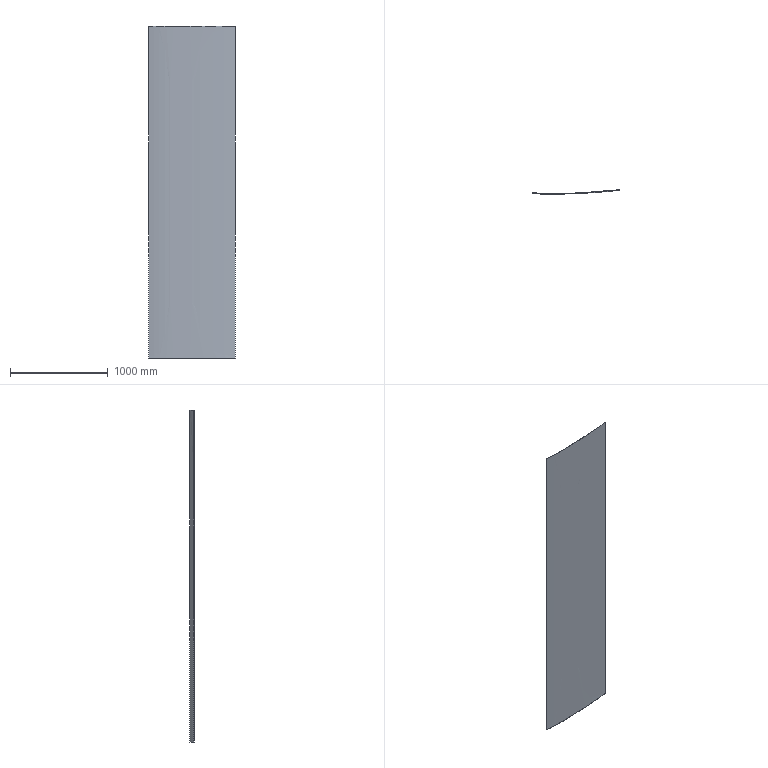Component | NX | SKIN_0_5_LOWER | 1 solid | 6 faces | box 887.13 x 42.02 x 3390 mm | volume 1497879 mm3 | plane 4 | other 2
STEP:
#1=CARTESIAN_POINT('',(0.,0.,0.));
#2=DIRECTION('',(0.,0.,1.));
#3=DIRECTION('',(1.,0.,0.));
#4=AXIS2_PLACEMENT_3D('',#1,#2,#3);
#5=CARTESIAN_POINT('',(5772.888,4104.218,-3390.));
#6=VERTEX_POINT('',#5);
#7=CARTESIAN_POINT('',(5772.824,4103.722,-3390.));
#8=VERTEX_POINT('',#7);
#9=CARTESIAN_POINT('',(5772.888,4104.218,-3390.));
#10=DIRECTION('',(-0.1274,-0.9919,0.));
#11=VECTOR('',#10,1.);
#12=LINE('',#9,#11);
#13=CARTESIAN_POINT('',(5772.888,4104.218,-0.));
#14=DIRECTION('',(0.9919,-0.1274,0.));
#15=DIRECTION('',(0.1274,0.9919,0.));
#16=AXIS2_PLACEMENT_3D('',#13,#14,#15);
#17=PLANE('',#16);
#18=CARTESIAN_POINT('',(0.,-3390.));
#19=DIRECTION('',(-1.,0.));
#20=VECTOR('',#19,1.);
#21=LINE('',#18,#20);
#22=(GEOMETRIC_REPRESENTATION_CONTEXT(2)PARAMETRIC_REPRESENTATION_CONTEXT()REPRESENTATION_CONTEXT('',''));
#23=DEFINITIONAL_REPRESENTATION('',(#21),#22);
#24=PCURVE('',#17,#23);
#25=CARTESIAN_POINT('',(6216.882,4101.421,-3390.));
#26=DIRECTION('',(0.,0.,-1.));
#27=DIRECTION('',(-1.,0.001745,0.));
#28=AXIS2_PLACEMENT_3D('',#25,#26,#27);
#29=PLANE('',#28);
#30=CARTESIAN_POINT('',(443.998,2.021));
#31=DIRECTION('',(0.1256,-0.9921));
#32=VECTOR('',#31,1.);
#33=LINE('',#30,#32);
#34=(GEOMETRIC_REPRESENTATION_CONTEXT(2)PARAMETRIC_REPRESENTATION_CONTEXT()REPRESENTATION_CONTEXT('',''));
#35=DEFINITIONAL_REPRESENTATION('',(#33),#34);
#36=PCURVE('',#29,#35);
#37=SURFACE_CURVE('',#12,(#24,#36),.PCURVE_S1.);
#38=EDGE_CURVE('',#6,#8,#37,.T.);
#39=ORIENTED_EDGE('',*,*,#38,.T.);
#40=CARTESIAN_POINT('',(5772.824,4103.722,-0.));
#41=VERTEX_POINT('',#40);
#42=CARTESIAN_POINT('',(5772.824,4103.722,-0.));
#43=DIRECTION('',(0.,0.,-1.));
#44=VECTOR('',#43,1.);
#45=LINE('',#42,#44);
#46=CARTESIAN_POINT('',(-0.5,0.));
#47=DIRECTION('',(0.,-1.));
#48=VECTOR('',#47,1.);
#49=LINE('',#46,#48);
#50=(GEOMETRIC_REPRESENTATION_CONTEXT(2)PARAMETRIC_REPRESENTATION_CONTEXT()REPRESENTATION_CONTEXT('',''));
#51=DEFINITIONAL_REPRESENTATION('',(#49),#50);
#52=PCURVE('',#17,#51);
#53=CARTESIAN_POINT('',(5772.824,4103.722,0.));
#54=CARTESIAN_POINT('',(5846.499,4094.26,0.));
#55=CARTESIAN_POINT('',(5920.588,4093.032,0.));
#56=CARTESIAN_POINT('',(6013.234,4094.576,0.));
#57=CARTESIAN_POINT('',(6031.765,4095.038,0.));
#58=CARTESIAN_POINT('',(6059.554,4095.829,0.));
#59=CARTESIAN_POINT('',(6068.816,4096.107,0.));
#60=CARTESIAN_POINT('',(6087.337,4096.677,0.));
#61=CARTESIAN_POINT('',(6133.632,4098.144,0.));
#62=CARTESIAN_POINT('',(6179.893,4099.843,0.));
#63=CARTESIAN_POINT('',(6364.839,4107.736,0.));
#64=CARTESIAN_POINT('',(6512.48,4117.559,0.));
#65=CARTESIAN_POINT('',(6659.952,4135.396,0.));
#66=B_SPLINE_CURVE_WITH_KNOTS('',3,(#53,#54,#55,#56,#57,#58,#59,#60,#61,#62,#63,#64,#65),.UNSPECIFIED.,.F.,.F.,(4,2,2,2,1,2,4),(0.,0.25,0.3125,0.3438,0.375,0.5,1.),.UNSPECIFIED.);
#67=DIRECTION('',(0.,0.,-1.));
#68=VECTOR('',#67,1.);
#69=SURFACE_OF_LINEAR_EXTRUSION('',#66,#68);
#70=CARTESIAN_POINT('',(-0.,0.));
#71=DIRECTION('',(0.,1.));
#72=VECTOR('',#71,1.);
#73=LINE('',#70,#72);
#74=(GEOMETRIC_REPRESENTATION_CONTEXT(2)PARAMETRIC_REPRESENTATION_CONTEXT()REPRESENTATION_CONTEXT('',''));
#75=DEFINITIONAL_REPRESENTATION('',(#73),#74);
#76=PCURVE('',#69,#75);
#77=SURFACE_CURVE('',#45,(#52,#76),.PCURVE_S1.);
#78=EDGE_CURVE('',#41,#8,#77,.T.);
#79=ORIENTED_EDGE('',*,*,#78,.F.);
#80=CARTESIAN_POINT('',(5772.888,4104.218,-0.));
#81=VERTEX_POINT('',#80);
#82=CARTESIAN_POINT('',(5772.888,4104.218,-0.));
#83=DIRECTION('',(-0.1274,-0.9919,0.));
#84=VECTOR('',#83,1.);
#85=LINE('',#82,#84);
#86=CARTESIAN_POINT('',(0.,0.));
#87=DIRECTION('',(-1.,0.));
#88=VECTOR('',#87,1.);
#89=LINE('',#86,#88);
#90=(GEOMETRIC_REPRESENTATION_CONTEXT(2)PARAMETRIC_REPRESENTATION_CONTEXT()REPRESENTATION_CONTEXT('',''));
#91=DEFINITIONAL_REPRESENTATION('',(#89),#90);
#92=PCURVE('',#17,#91);
#93=CARTESIAN_POINT('',(6216.882,4101.421,0.));
#94=DIRECTION('',(0.,0.,-1.));
#95=DIRECTION('',(-1.,0.001745,0.));
#96=AXIS2_PLACEMENT_3D('',#93,#94,#95);
#97=PLANE('',#96);
#98=CARTESIAN_POINT('',(443.998,2.021));
#99=DIRECTION('',(0.1256,-0.9921));
#100=VECTOR('',#99,1.);
#101=LINE('',#98,#100);
#102=(GEOMETRIC_REPRESENTATION_CONTEXT(2)PARAMETRIC_REPRESENTATION_CONTEXT()REPRESENTATION_CONTEXT('',''));
#103=DEFINITIONAL_REPRESENTATION('',(#101),#102);
#104=PCURVE('',#97,#103);
#105=SURFACE_CURVE('',#85,(#92,#104),.PCURVE_S1.);
#106=EDGE_CURVE('',#81,#41,#105,.T.);
#107=ORIENTED_EDGE('',*,*,#106,.F.);
#108=CARTESIAN_POINT('',(5772.888,4104.218,-0.));
#109=DIRECTION('',(0.,0.,-1.));
#110=VECTOR('',#109,1.);
#111=LINE('',#108,#110);
#112=CARTESIAN_POINT('',(0.,0.));
#113=DIRECTION('',(0.,-1.));
#114=VECTOR('',#113,1.);
#115=LINE('',#112,#114);
#116=(GEOMETRIC_REPRESENTATION_CONTEXT(2)PARAMETRIC_REPRESENTATION_CONTEXT()REPRESENTATION_CONTEXT('',''));
#117=DEFINITIONAL_REPRESENTATION('',(#115),#116);
#118=PCURVE('',#17,#117);
#119=CARTESIAN_POINT('',(6659.892,4135.892,-0.));
#120=CARTESIAN_POINT('',(6463.767,4112.17,-0.));
#121=CARTESIAN_POINT('',(6168.395,4097.815,-0.));
#122=CARTESIAN_POINT('',(5871.551,4091.547,-0.));
#123=CARTESIAN_POINT('',(5772.888,4104.218,-0.));
#124=B_SPLINE_CURVE_WITH_KNOTS('',3,(#119,#120,#121,#122,#123),.UNSPECIFIED.,.F.,.F.,(4,1,4),(0.,0.665,1.),.UNSPECIFIED.);
#125=DIRECTION('',(0.,0.,-1.));
#126=VECTOR('',#125,1.);
#127=SURFACE_OF_LINEAR_EXTRUSION('',#124,#126);
#128=CARTESIAN_POINT('',(1.,0.));
#129=DIRECTION('',(-0.,1.));
#130=VECTOR('',#129,1.);
#131=LINE('',#128,#130);
#132=(GEOMETRIC_REPRESENTATION_CONTEXT(2)PARAMETRIC_REPRESENTATION_CONTEXT()REPRESENTATION_CONTEXT('',''));
#133=DEFINITIONAL_REPRESENTATION('',(#131),#132);
#134=PCURVE('',#127,#133);
#135=SURFACE_CURVE('',#111,(#118,#134),.PCURVE_S1.);
#136=EDGE_CURVE('',#81,#6,#135,.T.);
#137=ORIENTED_EDGE('',*,*,#136,.T.);
#138=EDGE_LOOP('',(#39,#79,#107,#137));
#139=FACE_BOUND('',#138,.T.);
#140=ADVANCED_FACE('',(#139),#17,.F.);
#141=ORIENTED_EDGE('',*,*,#78,.F.);
#142=CARTESIAN_POINT('',(6659.952,4135.396,0.));
#143=VERTEX_POINT('',#142);
#144=CARTESIAN_POINT('',(5772.824,4103.722,0.));
#145=CARTESIAN_POINT('',(5846.499,4094.26,0.));
#146=CARTESIAN_POINT('',(5920.588,4093.032,0.));
#147=CARTESIAN_POINT('',(6013.234,4094.576,0.));
#148=CARTESIAN_POINT('',(6031.765,4095.038,0.));
#149=CARTESIAN_POINT('',(6059.554,4095.829,0.));
#150=CARTESIAN_POINT('',(6068.816,4096.107,0.));
#151=CARTESIAN_POINT('',(6087.337,4096.677,0.));
#152=CARTESIAN_POINT('',(6133.632,4098.144,0.));
#153=CARTESIAN_POINT('',(6179.893,4099.843,0.));
#154=CARTESIAN_POINT('',(6364.839,4107.736,0.));
#155=CARTESIAN_POINT('',(6512.48,4117.559,0.));
#156=CARTESIAN_POINT('',(6659.952,4135.396,0.));
#157=B_SPLINE_CURVE_WITH_KNOTS('',3,(#144,#145,#146,#147,#148,#149,#150,#151,#152,#153,#154,#155,#156),.UNSPECIFIED.,.F.,.F.,(4,2,2,2,1,2,4),(0.,0.25,0.3125,0.3438,0.375,0.5,1.),.UNSPECIFIED.);
#158=CARTESIAN_POINT('',(-0.,0.));
#159=DIRECTION('',(1.,0.));
#160=VECTOR('',#159,1.);
#161=LINE('',#158,#160);
#162=(GEOMETRIC_REPRESENTATION_CONTEXT(2)PARAMETRIC_REPRESENTATION_CONTEXT()REPRESENTATION_CONTEXT('',''));
#163=DEFINITIONAL_REPRESENTATION('',(#161),#162);
#164=PCURVE('',#69,#163);
#165=CARTESIAN_POINT('',(444.061,1.525));
#166=CARTESIAN_POINT('',(370.371,-7.808));
#167=CARTESIAN_POINT('',(296.279,-8.907));
#168=CARTESIAN_POINT('',(203.636,-7.201));
#169=CARTESIAN_POINT('',(185.106,-6.706));
#170=CARTESIAN_POINT('',(157.318,-5.867));
#171=CARTESIAN_POINT('',(148.057,-5.573));
#172=CARTESIAN_POINT('',(129.537,-4.97));
#173=CARTESIAN_POINT('',(83.244,-3.423));
#174=CARTESIAN_POINT('',(36.986,-1.643));
#175=CARTESIAN_POINT('',(-147.945,6.572));
#176=CARTESIAN_POINT('',(-295.569,16.653));
#177=CARTESIAN_POINT('',(-443.01,34.747));
#178=B_SPLINE_CURVE_WITH_KNOTS('',3,(#165,#166,#167,#168,#169,#170,#171,#172,#173,#174,#175,#176,#177),.UNSPECIFIED.,.F.,.F.,(4,2,2,2,1,2,4),(0.,0.25,0.3125,0.3438,0.375,0.5,1.),.UNSPECIFIED.);
#179=(GEOMETRIC_REPRESENTATION_CONTEXT(2)PARAMETRIC_REPRESENTATION_CONTEXT()REPRESENTATION_CONTEXT('',''));
#180=DEFINITIONAL_REPRESENTATION('',(#178),#179);
#181=PCURVE('',#97,#180);
#182=SURFACE_CURVE('',#157,(#164,#181),.PCURVE_S1.);
#183=EDGE_CURVE('',#41,#143,#182,.T.);
#184=ORIENTED_EDGE('',*,*,#183,.T.);
#185=CARTESIAN_POINT('',(6659.952,4135.396,-3390.));
#186=VERTEX_POINT('',#185);
#187=CARTESIAN_POINT('',(6659.952,4135.396,0.));
#188=DIRECTION('',(0.,0.,-1.));
#189=VECTOR('',#188,1.);
#190=LINE('',#187,#189);
#191=CARTESIAN_POINT('',(1.,0.));
#192=DIRECTION('',(0.,1.));
#193=VECTOR('',#192,1.);
#194=LINE('',#191,#193);
#195=(GEOMETRIC_REPRESENTATION_CONTEXT(2)PARAMETRIC_REPRESENTATION_CONTEXT()REPRESENTATION_CONTEXT('',''));
#196=DEFINITIONAL_REPRESENTATION('',(#194),#195);
#197=PCURVE('',#69,#196);
#198=CARTESIAN_POINT('',(6659.952,4135.396,-0.));
#199=DIRECTION('',(-0.9928,-0.1201,0.));
#200=DIRECTION('',(0.1201,-0.9928,0.));
#201=AXIS2_PLACEMENT_3D('',#198,#199,#200);
#202=PLANE('',#201);
#203=CARTESIAN_POINT('',(0.,0.));
#204=DIRECTION('',(0.,-1.));
#205=VECTOR('',#204,1.);
#206=LINE('',#203,#205);
#207=(GEOMETRIC_REPRESENTATION_CONTEXT(2)PARAMETRIC_REPRESENTATION_CONTEXT()REPRESENTATION_CONTEXT('',''));
#208=DEFINITIONAL_REPRESENTATION('',(#206),#207);
#209=PCURVE('',#202,#208);
#210=SURFACE_CURVE('',#190,(#197,#209),.PCURVE_S1.);
#211=EDGE_CURVE('',#143,#186,#210,.T.);
#212=ORIENTED_EDGE('',*,*,#211,.T.);
#213=CARTESIAN_POINT('',(5772.824,4103.722,-3390.));
#214=CARTESIAN_POINT('',(5846.499,4094.26,-3390.));
#215=CARTESIAN_POINT('',(5920.588,4093.032,-3390.));
#216=CARTESIAN_POINT('',(6013.234,4094.576,-3390.));
#217=CARTESIAN_POINT('',(6031.765,4095.038,-3390.));
#218=CARTESIAN_POINT('',(6059.554,4095.829,-3390.));
#219=CARTESIAN_POINT('',(6068.816,4096.107,-3390.));
#220=CARTESIAN_POINT('',(6087.337,4096.677,-3390.));
#221=CARTESIAN_POINT('',(6133.632,4098.144,-3390.));
#222=CARTESIAN_POINT('',(6179.893,4099.843,-3390.));
#223=CARTESIAN_POINT('',(6364.839,4107.736,-3390.));
#224=CARTESIAN_POINT('',(6512.48,4117.559,-3390.));
#225=CARTESIAN_POINT('',(6659.952,4135.396,-3390.));
#226=B_SPLINE_CURVE_WITH_KNOTS('',3,(#213,#214,#215,#216,#217,#218,#219,#220,#221,#222,#223,#224,#225),.UNSPECIFIED.,.F.,.F.,(4,2,2,2,1,2,4),(0.,0.25,0.3125,0.3438,0.375,0.5,1.),.UNSPECIFIED.);
#227=CARTESIAN_POINT('',(0.,3390.));
#228=DIRECTION('',(1.,0.));
#229=VECTOR('',#228,1.);
#230=LINE('',#227,#229);
#231=(GEOMETRIC_REPRESENTATION_CONTEXT(2)PARAMETRIC_REPRESENTATION_CONTEXT()REPRESENTATION_CONTEXT('',''));
#232=DEFINITIONAL_REPRESENTATION('',(#230),#231);
#233=PCURVE('',#69,#232);
#234=CARTESIAN_POINT('',(444.061,1.525));
#235=CARTESIAN_POINT('',(370.371,-7.808));
#236=CARTESIAN_POINT('',(296.279,-8.907));
#237=CARTESIAN_POINT('',(203.636,-7.201));
#238=CARTESIAN_POINT('',(185.106,-6.706));
#239=CARTESIAN_POINT('',(157.318,-5.867));
#240=CARTESIAN_POINT('',(148.057,-5.573));
#241=CARTESIAN_POINT('',(129.537,-4.97));
#242=CARTESIAN_POINT('',(83.244,-3.423));
#243=CARTESIAN_POINT('',(36.986,-1.643));
#244=CARTESIAN_POINT('',(-147.945,6.572));
#245=CARTESIAN_POINT('',(-295.569,16.653));
#246=CARTESIAN_POINT('',(-443.01,34.747));
#247=B_SPLINE_CURVE_WITH_KNOTS('',3,(#234,#235,#236,#237,#238,#239,#240,#241,#242,#243,#244,#245,#246),.UNSPECIFIED.,.F.,.F.,(4,2,2,2,1,2,4),(0.,0.25,0.3125,0.3438,0.375,0.5,1.),.UNSPECIFIED.);
#248=(GEOMETRIC_REPRESENTATION_CONTEXT(2)PARAMETRIC_REPRESENTATION_CONTEXT()REPRESENTATION_CONTEXT('',''));
#249=DEFINITIONAL_REPRESENTATION('',(#247),#248);
#250=PCURVE('',#29,#249);
#251=SURFACE_CURVE('',#226,(#233,#250),.PCURVE_S1.);
#252=EDGE_CURVE('',#8,#186,#251,.T.);
#253=ORIENTED_EDGE('',*,*,#252,.F.);
#254=EDGE_LOOP('',(#141,#184,#212,#253));
#255=FACE_BOUND('',#254,.F.);
#256=ADVANCED_FACE('',(#255),#69,.F.);
#257=CARTESIAN_POINT('',(6659.892,4135.892,-3390.));
#258=VERTEX_POINT('',#257);
#259=CARTESIAN_POINT('',(6659.952,4135.396,-3390.));
#260=DIRECTION('',(-0.1201,0.9928,0.));
#261=VECTOR('',#260,1.);
#262=LINE('',#259,#261);
#263=CARTESIAN_POINT('',(0.,-3390.));
#264=DIRECTION('',(-1.,0.));
#265=VECTOR('',#264,1.);
#266=LINE('',#263,#265);
#267=(GEOMETRIC_REPRESENTATION_CONTEXT(2)PARAMETRIC_REPRESENTATION_CONTEXT()REPRESENTATION_CONTEXT('',''));
#268=DEFINITIONAL_REPRESENTATION('',(#266),#267);
#269=PCURVE('',#202,#268);
#270=CARTESIAN_POINT('',(-443.01,34.747));
#271=DIRECTION('',(0.1218,0.9926));
#272=VECTOR('',#271,1.);
#273=LINE('',#270,#272);
#274=(GEOMETRIC_REPRESENTATION_CONTEXT(2)PARAMETRIC_REPRESENTATION_CONTEXT()REPRESENTATION_CONTEXT('',''));
#275=DEFINITIONAL_REPRESENTATION('',(#273),#274);
#276=PCURVE('',#29,#275);
#277=SURFACE_CURVE('',#262,(#269,#276),.PCURVE_S1.);
#278=EDGE_CURVE('',#186,#258,#277,.T.);
#279=ORIENTED_EDGE('',*,*,#278,.T.);
#280=CARTESIAN_POINT('',(6659.892,4135.892,-0.));
#281=VERTEX_POINT('',#280);
#282=CARTESIAN_POINT('',(6659.892,4135.892,-0.));
#283=DIRECTION('',(0.,0.,-1.));
#284=VECTOR('',#283,1.);
#285=LINE('',#282,#284);
#286=CARTESIAN_POINT('',(-0.5,0.));
#287=DIRECTION('',(0.,-1.));
#288=VECTOR('',#287,1.);
#289=LINE('',#286,#288);
#290=(GEOMETRIC_REPRESENTATION_CONTEXT(2)PARAMETRIC_REPRESENTATION_CONTEXT()REPRESENTATION_CONTEXT('',''));
#291=DEFINITIONAL_REPRESENTATION('',(#289),#290);
#292=PCURVE('',#202,#291);
#293=CARTESIAN_POINT('',(0.,0.));
#294=DIRECTION('',(-0.,1.));
#295=VECTOR('',#294,1.);
#296=LINE('',#293,#295);
#297=(GEOMETRIC_REPRESENTATION_CONTEXT(2)PARAMETRIC_REPRESENTATION_CONTEXT()REPRESENTATION_CONTEXT('',''));
#298=DEFINITIONAL_REPRESENTATION('',(#296),#297);
#299=PCURVE('',#127,#298);
#300=SURFACE_CURVE('',#285,(#292,#299),.PCURVE_S1.);
#301=EDGE_CURVE('',#281,#258,#300,.T.);
#302=ORIENTED_EDGE('',*,*,#301,.F.);
#303=CARTESIAN_POINT('',(6659.952,4135.396,-0.));
#304=DIRECTION('',(-0.1201,0.9928,0.));
#305=VECTOR('',#304,1.);
#306=LINE('',#303,#305);
#307=CARTESIAN_POINT('',(0.,0.));
#308=DIRECTION('',(-1.,0.));
#309=VECTOR('',#308,1.);
#310=LINE('',#307,#309);
#311=(GEOMETRIC_REPRESENTATION_CONTEXT(2)PARAMETRIC_REPRESENTATION_CONTEXT()REPRESENTATION_CONTEXT('',''));
#312=DEFINITIONAL_REPRESENTATION('',(#310),#311);
#313=PCURVE('',#202,#312);
#314=CARTESIAN_POINT('',(-443.01,34.747));
#315=DIRECTION('',(0.1218,0.9926));
#316=VECTOR('',#315,1.);
#317=LINE('',#314,#316);
#318=(GEOMETRIC_REPRESENTATION_CONTEXT(2)PARAMETRIC_REPRESENTATION_CONTEXT()REPRESENTATION_CONTEXT('',''));
#319=DEFINITIONAL_REPRESENTATION('',(#317),#318);
#320=PCURVE('',#97,#319);
#321=SURFACE_CURVE('',#306,(#313,#320),.PCURVE_S1.);
#322=EDGE_CURVE('',#143,#281,#321,.T.);
#323=ORIENTED_EDGE('',*,*,#322,.F.);
#324=ORIENTED_EDGE('',*,*,#211,.T.);
#325=EDGE_LOOP('',(#279,#302,#323,#324));
#326=FACE_BOUND('',#325,.T.);
#327=ADVANCED_FACE('',(#326),#202,.F.);
#328=ORIENTED_EDGE('',*,*,#301,.F.);
#329=CARTESIAN_POINT('',(6659.892,4135.892,-0.));
#330=CARTESIAN_POINT('',(6463.767,4112.17,-0.));
#331=CARTESIAN_POINT('',(6168.395,4097.815,-0.));
#332=CARTESIAN_POINT('',(5871.551,4091.547,-0.));
#333=CARTESIAN_POINT('',(5772.888,4104.218,-0.));
#334=B_SPLINE_CURVE_WITH_KNOTS('',3,(#329,#330,#331,#332,#333),.UNSPECIFIED.,.F.,.F.,(4,1,4),(0.,0.665,1.),.UNSPECIFIED.);
#335=CARTESIAN_POINT('',(0.,0.));
#336=DIRECTION('',(1.,0.));
#337=VECTOR('',#336,1.);
#338=LINE('',#335,#337);
#339=(GEOMETRIC_REPRESENTATION_CONTEXT(2)PARAMETRIC_REPRESENTATION_CONTEXT()REPRESENTATION_CONTEXT('',''));
#340=DEFINITIONAL_REPRESENTATION('',(#338),#339);
#341=PCURVE('',#127,#340);
#342=CARTESIAN_POINT('',(-442.949,35.244));
#343=CARTESIAN_POINT('',(-246.865,11.18));
#344=CARTESIAN_POINT('',(48.481,-3.691));
#345=CARTESIAN_POINT('',(345.313,-10.477));
#346=CARTESIAN_POINT('',(443.998,2.021));
#347=B_SPLINE_CURVE_WITH_KNOTS('',3,(#342,#343,#344,#345,#346),.UNSPECIFIED.,.F.,.F.,(4,1,4),(0.,0.665,1.),.UNSPECIFIED.);
#348=(GEOMETRIC_REPRESENTATION_CONTEXT(2)PARAMETRIC_REPRESENTATION_CONTEXT()REPRESENTATION_CONTEXT('',''));
#349=DEFINITIONAL_REPRESENTATION('',(#347),#348);
#350=PCURVE('',#97,#349);
#351=SURFACE_CURVE('',#334,(#341,#350),.PCURVE_S1.);
#352=EDGE_CURVE('',#281,#81,#351,.T.);
#353=ORIENTED_EDGE('',*,*,#352,.T.);
#354=ORIENTED_EDGE('',*,*,#136,.T.);
#355=CARTESIAN_POINT('',(6659.892,4135.892,-3390.));
#356=CARTESIAN_POINT('',(6463.767,4112.17,-3390.));
#357=CARTESIAN_POINT('',(6168.395,4097.815,-3390.));
#358=CARTESIAN_POINT('',(5871.551,4091.547,-3390.));
#359=CARTESIAN_POINT('',(5772.888,4104.218,-3390.));
#360=B_SPLINE_CURVE_WITH_KNOTS('',3,(#355,#356,#357,#358,#359),.UNSPECIFIED.,.F.,.F.,(4,1,4),(0.,0.665,1.),.UNSPECIFIED.);
#361=CARTESIAN_POINT('',(-0.,3390.));
#362=DIRECTION('',(1.,0.));
#363=VECTOR('',#362,1.);
#364=LINE('',#361,#363);
#365=(GEOMETRIC_REPRESENTATION_CONTEXT(2)PARAMETRIC_REPRESENTATION_CONTEXT()REPRESENTATION_CONTEXT('',''));
#366=DEFINITIONAL_REPRESENTATION('',(#364),#365);
#367=PCURVE('',#127,#366);
#368=CARTESIAN_POINT('',(-442.949,35.244));
#369=CARTESIAN_POINT('',(-246.865,11.18));
#370=CARTESIAN_POINT('',(48.481,-3.691));
#371=CARTESIAN_POINT('',(345.313,-10.477));
#372=CARTESIAN_POINT('',(443.998,2.021));
#373=B_SPLINE_CURVE_WITH_KNOTS('',3,(#368,#369,#370,#371,#372),.UNSPECIFIED.,.F.,.F.,(4,1,4),(0.,0.665,1.),.UNSPECIFIED.);
#374=(GEOMETRIC_REPRESENTATION_CONTEXT(2)PARAMETRIC_REPRESENTATION_CONTEXT()REPRESENTATION_CONTEXT('',''));
#375=DEFINITIONAL_REPRESENTATION('',(#373),#374);
#376=PCURVE('',#29,#375);
#377=SURFACE_CURVE('',#360,(#367,#376),.PCURVE_S1.);
#378=EDGE_CURVE('',#258,#6,#377,.T.);
#379=ORIENTED_EDGE('',*,*,#378,.F.);
#380=EDGE_LOOP('',(#328,#353,#354,#379));
#381=FACE_BOUND('',#380,.F.);
#382=ADVANCED_FACE('',(#381),#127,.F.);
#383=ORIENTED_EDGE('',*,*,#106,.T.);
#384=ORIENTED_EDGE('',*,*,#183,.T.);
#385=ORIENTED_EDGE('',*,*,#322,.T.);
#386=ORIENTED_EDGE('',*,*,#352,.T.);
#387=EDGE_LOOP('',(#383,#384,#385,#386));
#388=FACE_BOUND('',#387,.T.);
#389=ADVANCED_FACE('',(#388),#97,.F.);
#390=ORIENTED_EDGE('',*,*,#38,.F.);
#391=ORIENTED_EDGE('',*,*,#378,.F.);
#392=ORIENTED_EDGE('',*,*,#278,.F.);
#393=ORIENTED_EDGE('',*,*,#252,.F.);
#394=EDGE_LOOP('',(#390,#391,#392,#393));
#395=FACE_BOUND('',#394,.T.);
#396=ADVANCED_FACE('',(#395),#29,.T.);
#397=CLOSED_SHELL('',(#140,#256,#327,#382,#389,#396));
#398=MANIFOLD_SOLID_BREP('',#397);
#399=(LENGTH_UNIT()NAMED_UNIT(*)SI_UNIT(.MILLI.,.METRE.));
#400=UNCERTAINTY_MEASURE_WITH_UNIT(LENGTH_MEASURE(0.0000001),#399,'','');
#401=(NAMED_UNIT(*)PLANE_ANGLE_UNIT()SI_UNIT($,.RADIAN.));
#402=(NAMED_UNIT(*)SI_UNIT($,.STERADIAN.)SOLID_ANGLE_UNIT());
#403=(GEOMETRIC_REPRESENTATION_CONTEXT(3)GLOBAL_UNCERTAINTY_ASSIGNED_CONTEXT((#400))GLOBAL_UNIT_ASSIGNED_CONTEXT((#399,#401,#402))REPRESENTATION_CONTEXT('',''));
#404=ADVANCED_BREP_SHAPE_REPRESENTATION('',(#4,#398),#403);